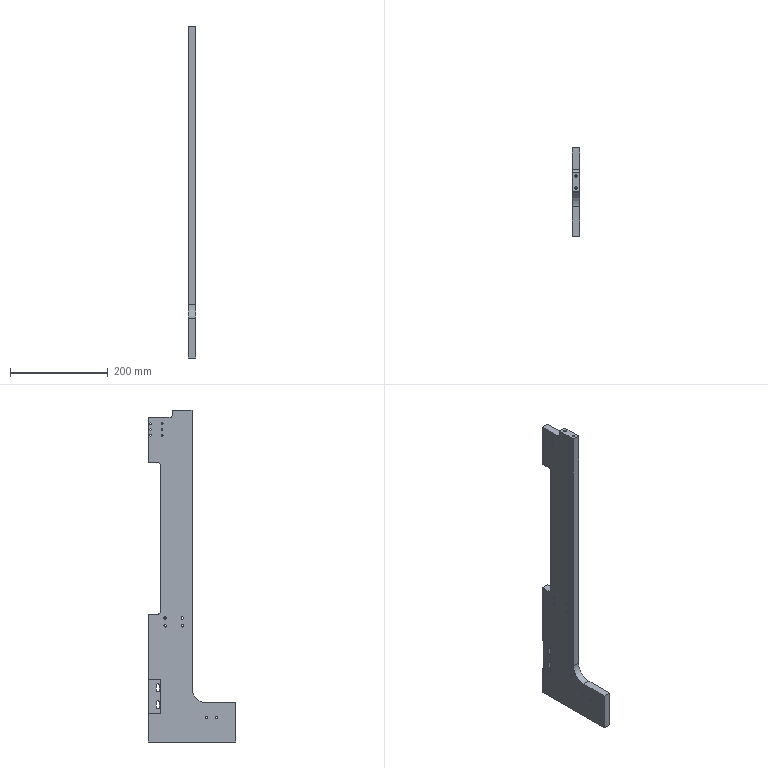Component | SolidWorks | 30-28A-1 | 1 solid | 110 faces | box 15 x 180 x 680 mm | volume 887754 mm3 | cylinder 62 | plane 28 | cone 20 | commonest cylinder face diameters 5 x22 3.3 x16 11 x6 6.6 x6 3 x4 10 x3 8.1 x2 4 x2
build123d program:
from build123d import *

# Parameters (mm, degrees)
EXTRUDE1_DEPTH        = 15
LINEAR_PATTERN2_COUNT = 4
LINEAR_PATTERN2_PITCH = 140
M8_TAPPED_HOLE1_D     = 8.1
M8_TAPPED_HOLE1_DEPTH = 36.25
M8_TAPPED_HOLE1_TIP   = 2.433
M6_TAPPED_HOLE2_D     = 5
M6_TAPPED_HOLE2_DEPTH = 17
M6_TAPPED_HOLE2_TIP   = 1.502
M6_TAPPED_HOLE1_D     = 5
M6_TAPPED_HOLE1_DEPTH = 17
M6_TAPPED_HOLE1_TIP   = 1.502
SKETCH35_W            = 310
SKETCH35_H            = 25
CUT_EXTRUDE1_DEPTH    = 704.58
FILLET1_R             = 5
M4_TAPPED_HOLE5_D     = 3.3
M6_TAPPED_HOLE3_D     = 5
CUT_EXTRUDE3_DEPTH    = 704.58
SKETCH43_R            = 1.5
CUT_EXTRUDE4_DEPTH    = 704.58
M6_TAPPED_HOLE4_D     = 5
CUT_EXTRUDE6_DEPTH    = 704.58
CUT_EXTRUDE7_DEPTH    = 2
CUT_EXTRUDE8_DEPTH    = 6


with BuildPart() as part:
    # Sketch1 → Extrude1 (new body)
    with BuildSketch(Plane.XY):
        with BuildLine():
            Line((0, 0), (0, 180))
            Line((0, 180), (680, 180))
            Line((680, 180), (680, 90))
            Line((680, 90), (110, 90))
            ThreePointArc((110, 90), (88.787, 81.213), (80, 60))
            Line((80, 60), (80, 0))
            Line((80, 0), (0, 0))
        make_face()
    extrude(amount=EXTRUDE1_DEPTH)

    # Sketch4 → M4 Tapped Hole1 (revolve, cut)
    with BuildSketch(Plane(origin=(100, 127.5, 0), x_dir=(0, 1, 0), z_dir=(1, 0, 0))):
        Polygon((0, 0), (0, 12.491), (1.65, 11.5), (1.65, 0), align=None)
    m4_tapped_hole1 = revolve(axis=Axis((100, 127.5, -6.35), (0, 0, 1)), mode=Mode.SUBTRACT)

    # Linear Pattern2: M4 Tapped Hole1 ×4
    with Locations(*[(i * LINEAR_PATTERN2_PITCH, 0, 0) for i in range(1, LINEAR_PATTERN2_COUNT)]):
        add(m4_tapped_hole1, mode=Mode.SUBTRACT)

    # M8 Tapped Hole1
    with Locations(Plane(origin=(0, 180, 0), x_dir=(-1, 0, 0), z_dir=(0, 1, 0))):
        with Locations((-50, 7.5)):
            Hole(M8_TAPPED_HOLE1_D / 2, depth=M8_TAPPED_HOLE1_DEPTH)
            with Locations((0, 0, -(M8_TAPPED_HOLE1_DEPTH + M8_TAPPED_HOLE1_TIP / 2))):  # 118° drill point
                Cone(0, M8_TAPPED_HOLE1_D / 2, M8_TAPPED_HOLE1_TIP, mode=Mode.SUBTRACT)

    # M6 Tapped Hole2
    with Locations(Plane(origin=(680, 0, 0), x_dir=(0, 0, -1), z_dir=(1, 0, 0))):
        with Locations((-7.5, 122), (-7.5, 98)):
            Hole(M6_TAPPED_HOLE2_D / 2, depth=M6_TAPPED_HOLE2_DEPTH)
            with Locations((0, 0, -(M6_TAPPED_HOLE2_DEPTH + M6_TAPPED_HOLE2_TIP / 2))):  # 118° drill point
                Cone(0, M6_TAPPED_HOLE2_D / 2, M6_TAPPED_HOLE2_TIP, mode=Mode.SUBTRACT)

    # M6 Tapped Hole1
    with Locations(Plane.ZY):
        with Locations((7.5, 90), (7.5, 15), (7.5, 165)):
            Hole(M6_TAPPED_HOLE1_D / 2, depth=M6_TAPPED_HOLE1_DEPTH)
            with Locations((0, 0, -(M6_TAPPED_HOLE1_DEPTH + M6_TAPPED_HOLE1_TIP / 2))):  # 118° drill point
                Cone(0, M6_TAPPED_HOLE1_D / 2, M6_TAPPED_HOLE1_TIP, mode=Mode.SUBTRACT)

    # Sketch35 → Cut-Extrude1 (cut, through all)
    with BuildSketch(Plane(origin=(0, 0, 0), x_dir=(-1, 0, 0), z_dir=(0, 0, -1))):
        with Locations((-417, 167.5)):
            Rectangle(SKETCH35_W, SKETCH35_H)
    extrude(amount=-CUT_EXTRUDE1_DEPTH, mode=Mode.SUBTRACT)

    # Fillet1
    fillet1_edges = [part.edges().sort_by_distance(p)[0] for p in [
        (572, 155, 7.5),
        (262, 155, 7.5),
    ]]
    fillet(fillet1_edges, radius=FILLET1_R)

    # M4 Tapped Hole5 (through all)
    with Locations(Plane(origin=(0, 0, 0), x_dir=(-1, 0, 0), z_dir=(0, 0, -1))):
        with Locations((-652, 175), (-628, 175), (-628, 151), (-652, 151)):
            Hole(M4_TAPPED_HOLE5_D / 2)

    # M6 Tapped Hole3 (through all)
    with Locations(Plane(origin=(0, 0, 0), x_dir=(-1, 0, 0), z_dir=(0, 0, -1))):
        with Locations((-254, 145), (-238, 145), (-254, 110), (-238, 110)):
            Hole(M6_TAPPED_HOLE3_D / 2)

    # Sketch45 → Cut-Extrude3 (cut, through all)
    with BuildSketch(Plane(origin=(0, 0, 0), x_dir=(-1, 0, 0), z_dir=(0, 0, -1))):
        with BuildLine():
            Line((-116, 163.3), (-106, 163.3))
            ThreePointArc((-106, 163.3), (-102.7, 160), (-106, 156.7))
            Line((-106, 156.7), (-116, 156.7))
            ThreePointArc((-116, 156.7), (-119.3, 160), (-116, 163.3))
        make_face()
        with BuildLine():
            Line((-71, 156.7), (-81, 156.7))
            ThreePointArc((-81, 156.7), (-84.3, 160), (-81, 163.3))
            Line((-81, 163.3), (-71, 163.3))
            ThreePointArc((-71, 163.3), (-67.7, 160), (-71, 156.7))
        make_face()
    extrude(amount=-CUT_EXTRUDE3_DEPTH, mode=Mode.SUBTRACT)

    # Sketch43 → Cut-Extrude4 (cut, through all)
    with BuildSketch(Plane(origin=(0, 0, 0), x_dir=(-1, 0, 0), z_dir=(0, 0, -1))):
        with Locations((-640, 175)):
            Circle(SKETCH43_R)
        with Locations((-640, 151)):
            Circle(SKETCH43_R)
    extrude(amount=-CUT_EXTRUDE4_DEPTH, mode=Mode.SUBTRACT)

    # M6 Tapped Hole4 (through all)
    with Locations(Plane(origin=(0, 0, 0), x_dir=(-1, 0, 0), z_dir=(0, 0, -1))):
        with Locations((-50, 60), (-50, 40)):
            Hole(M6_TAPPED_HOLE4_D / 2)

    # Sketch51 → Cut-Extrude6 (cut, through all)
    with BuildSketch(Plane(origin=(0, 0, 0), x_dir=(-1, 0, 0), z_dir=(0, 0, -1))):
        with BuildLine():
            Line((-680, 180), (-665, 180))
            Line((-665, 180), (-665, 135))
            ThreePointArc((-665, 135), (-666.464, 131.464), (-670, 130))
            Line((-670, 130), (-680, 130))
            Line((-680, 130), (-680, 180))
        make_face()
    extrude(amount=-CUT_EXTRUDE6_DEPTH, mode=Mode.SUBTRACT)

    # Sketch52 → Cut-Extrude7 (cut)
    with BuildSketch(Plane.XY.offset(15)):
        with BuildLine():
            Line((58.5, 180), (128.5, 180))
            Line((128.5, 180), (128.5, 157))
            ThreePointArc((128.5, 157), (127.914, 155.586), (126.5, 155))
            Line((126.5, 155), (60.5, 155))
            ThreePointArc((60.5, 155), (59.086, 155.586), (58.5, 157))
            Line((58.5, 157), (58.5, 180))
        make_face()
    extrude(amount=-CUT_EXTRUDE7_DEPTH, mode=Mode.SUBTRACT)

    # Sketch53 → Cut-Extrude8 (cut)
    # profile 1 of 2: a face of its own
    with BuildSketch(Plane(origin=(0, 0, 0), x_dir=(-1, 0, 0), z_dir=(0, 0, -1))):
        with BuildLine():
            Line((-116, 154.5), (-106, 154.5))
            ThreePointArc((-106, 154.5), (-100.5, 160), (-106, 165.5))
            Line((-106, 165.5), (-116, 165.5))
            ThreePointArc((-116, 165.5), (-121.5, 160), (-116, 154.5))
        make_face()
        with BuildLine():
            Line((-116, 156.7), (-106, 156.7))
            ThreePointArc((-106, 156.7), (-102.7, 160), (-106, 163.3))
            Line((-106, 163.3), (-116, 163.3))
            ThreePointArc((-116, 163.3), (-119.3, 160), (-116, 156.7))
        make_face(mode=Mode.SUBTRACT)
    # profile 2 of 2: a face of its own
    with BuildSketch(Plane(origin=(0, 0, 0), x_dir=(-1, 0, 0), z_dir=(0, 0, -1))):
        with BuildLine():
            Line((-81, 154.5), (-71, 154.5))
            ThreePointArc((-71, 154.5), (-65.5, 160), (-71, 165.5))
            Line((-71, 165.5), (-81, 165.5))
            ThreePointArc((-81, 165.5), (-86.5, 160), (-81, 154.5))
        make_face()
        with BuildLine():
            Line((-81, 156.7), (-71, 156.7))
            ThreePointArc((-71, 156.7), (-67.7, 160), (-71, 163.3))
            Line((-71, 163.3), (-81, 163.3))
            ThreePointArc((-81, 163.3), (-84.3, 160), (-81, 156.7))
        make_face(mode=Mode.SUBTRACT)
    extrude(amount=-CUT_EXTRUDE8_DEPTH, mode=Mode.SUBTRACT)


solid = part.part

# Placed as in the assembly
solid = solid.moved(Location((-429.208, -167.092, 39.188), (0, -90, 0)))